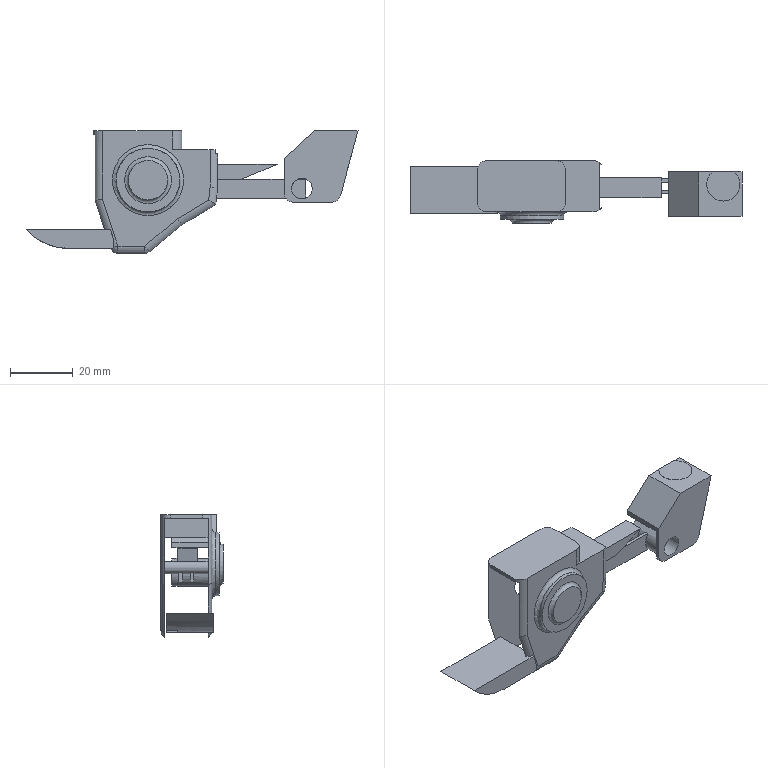Component | NX | OUTER_HUB_3 | 1 solid | 103 faces | volume 8768 mm3 | plane 72 | cylinder 25 | sphere 4 | torus 2 | commonest cylinder face diameters 6 x18 3.86 x1 6.599 x1 8.999 x1 10.549 x1 20.267 x1 35.858 x1 10.2 x1